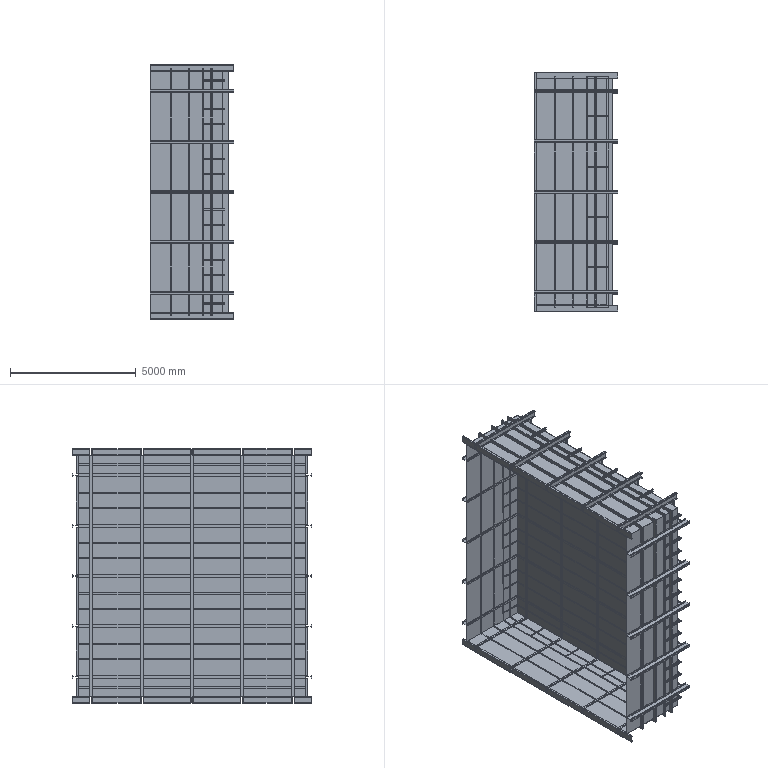Assembly | NX | mm | 87 component files | 280 solids | 3021 faces | box 3300 x 9500 x 10100 mm | volume 2362847389 mm3 | plane 3021
Bill of materials:
unnamed part 1 | 5 |  | Long straight prismatic member with an H/wide-flange cross-section (two parallel flanges joined by a central web); appears as one continuous body.
unnamed part 2 | 20 |  | Long straight I-section beam with a section deeper than its flanges are wide, and a thin web; appears as one continuous body.
unnamed part 3 | 5 |  | H/wide-flange profile split along its length into six separate collinear segments (two short end pieces and four longer, roughly equal middle pieces) separated by small gaps.
unnamed part 4 | 2 |  | C/channel section (web with two flanges on one side) split along its length into six collinear segments: two short end pieces and four longer middle pieces with small gaps between them.
unnamed part 5 | 8 |  | C/channel section split into six collinear segments (shorter at both ends, four longer in the middle). The channel flanges are relatively wide compared with the web depth.
unnamed part 6 | 28 |  | Short C/channel section made of two collinear segments, one shorter than the other, separated by a gap.
unnamed part 7 | 1 |  | Plain rectangular solid block or thick plate with flat faces and sharp edges.
unnamed part 8 | 18 |  | Shallow U-channel profile with a wide web and two thick upright legs, split along its length into six collinear segments (short end pieces and four longer middle pieces).
Mates:
1. touch align | chunshuijincao_caogang3 15 face | chunshuijincao_caogang1 1 face
2. touch align | chunshuijincao_caogang3 19 face | chunshuijincao_caogang1 1 face